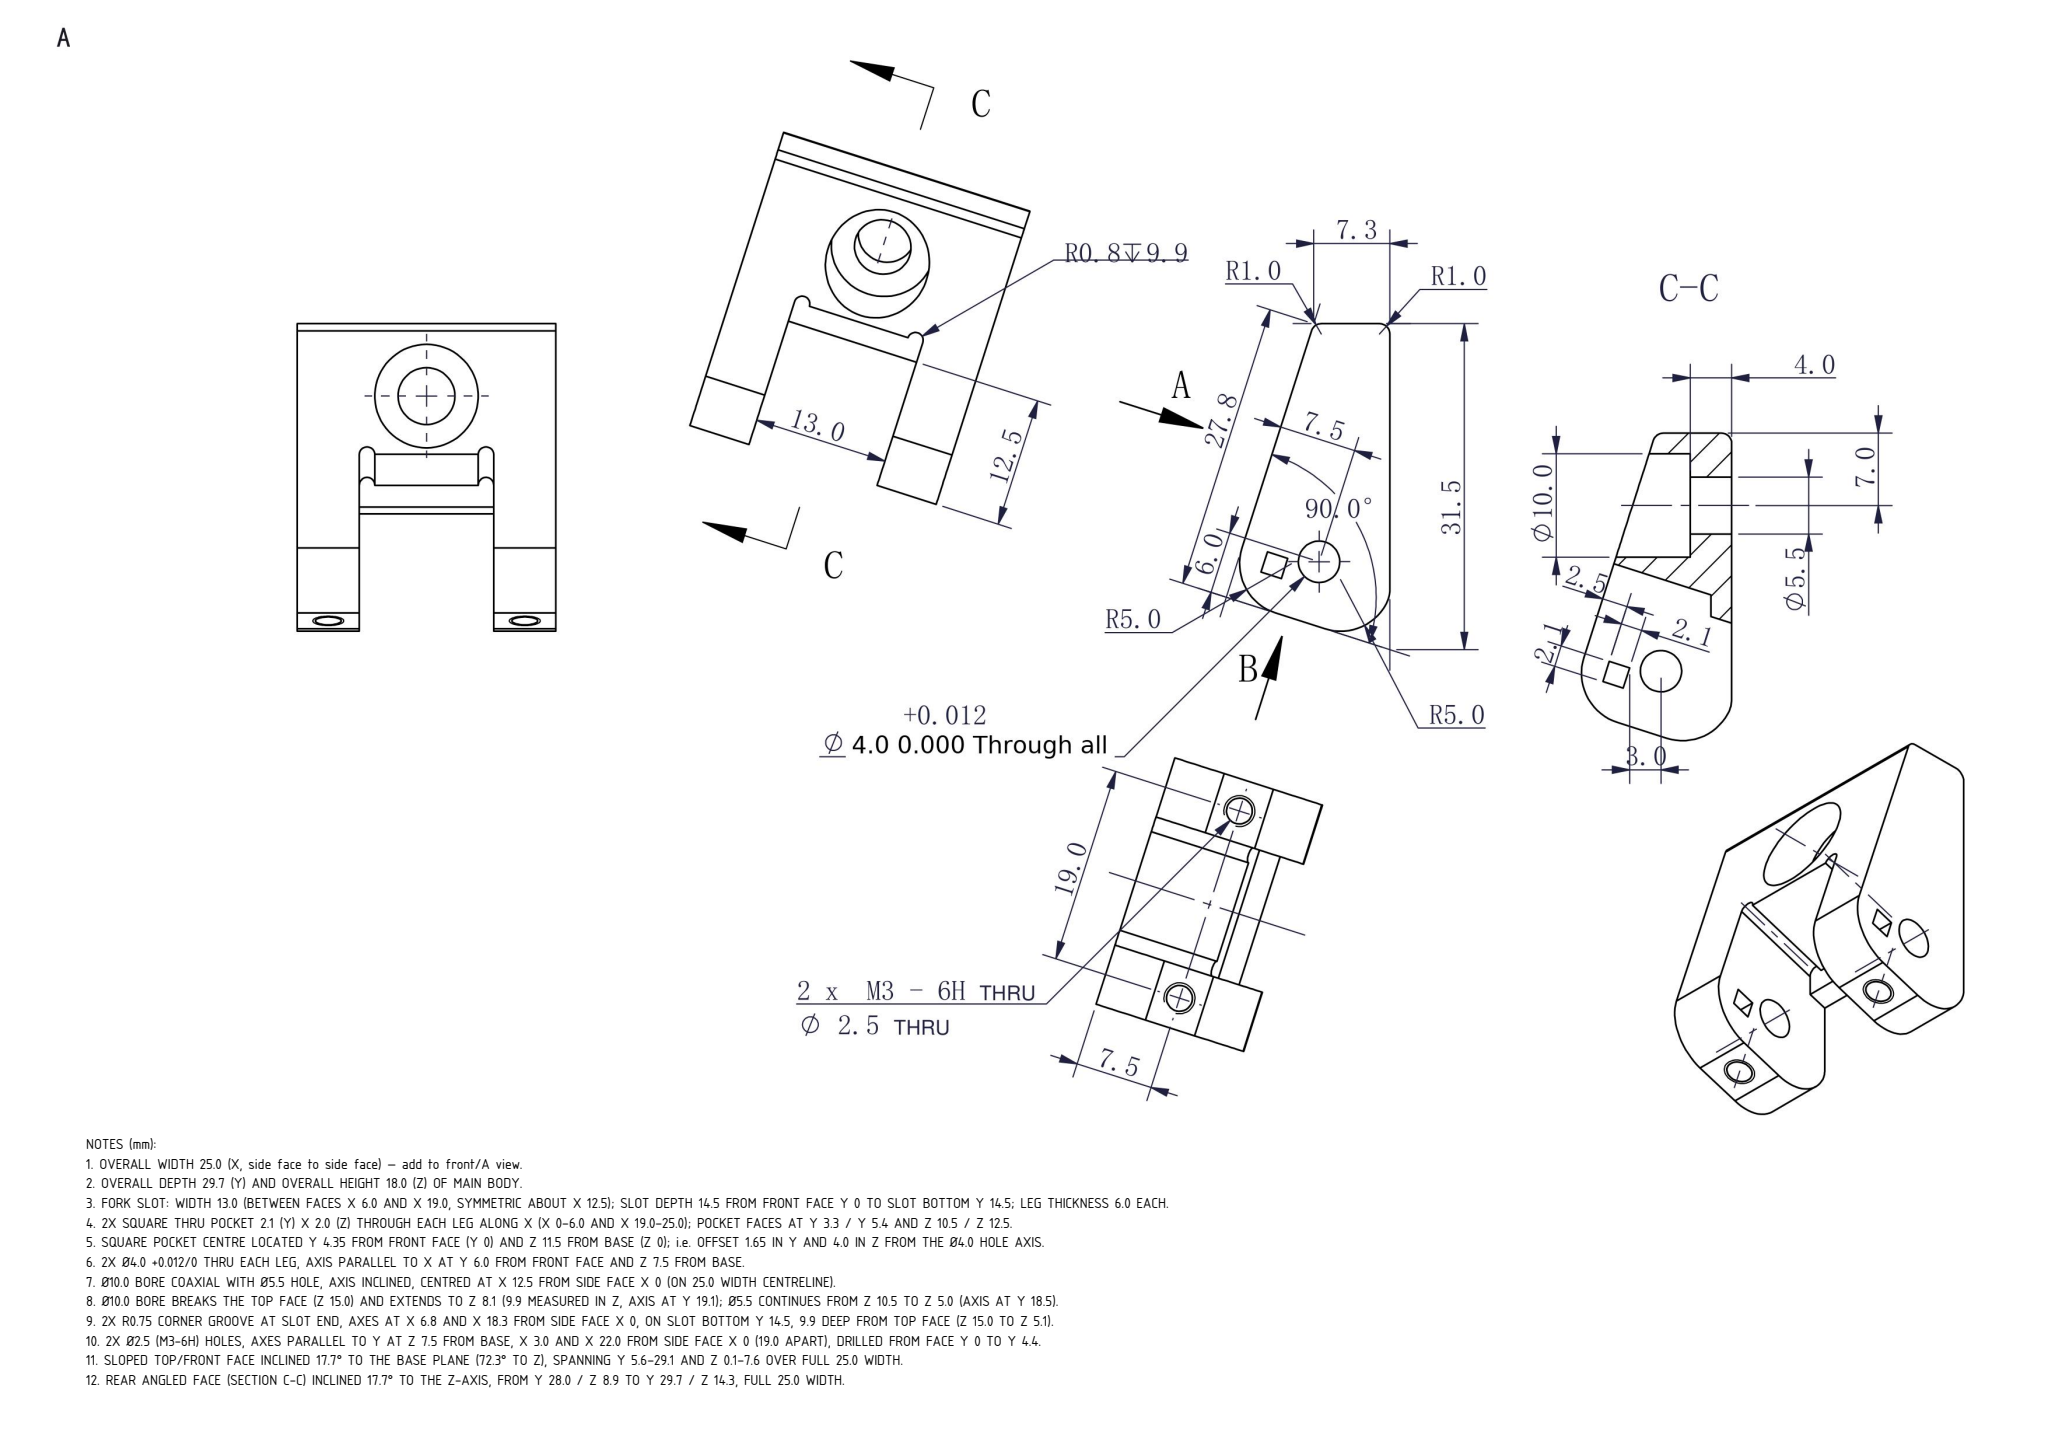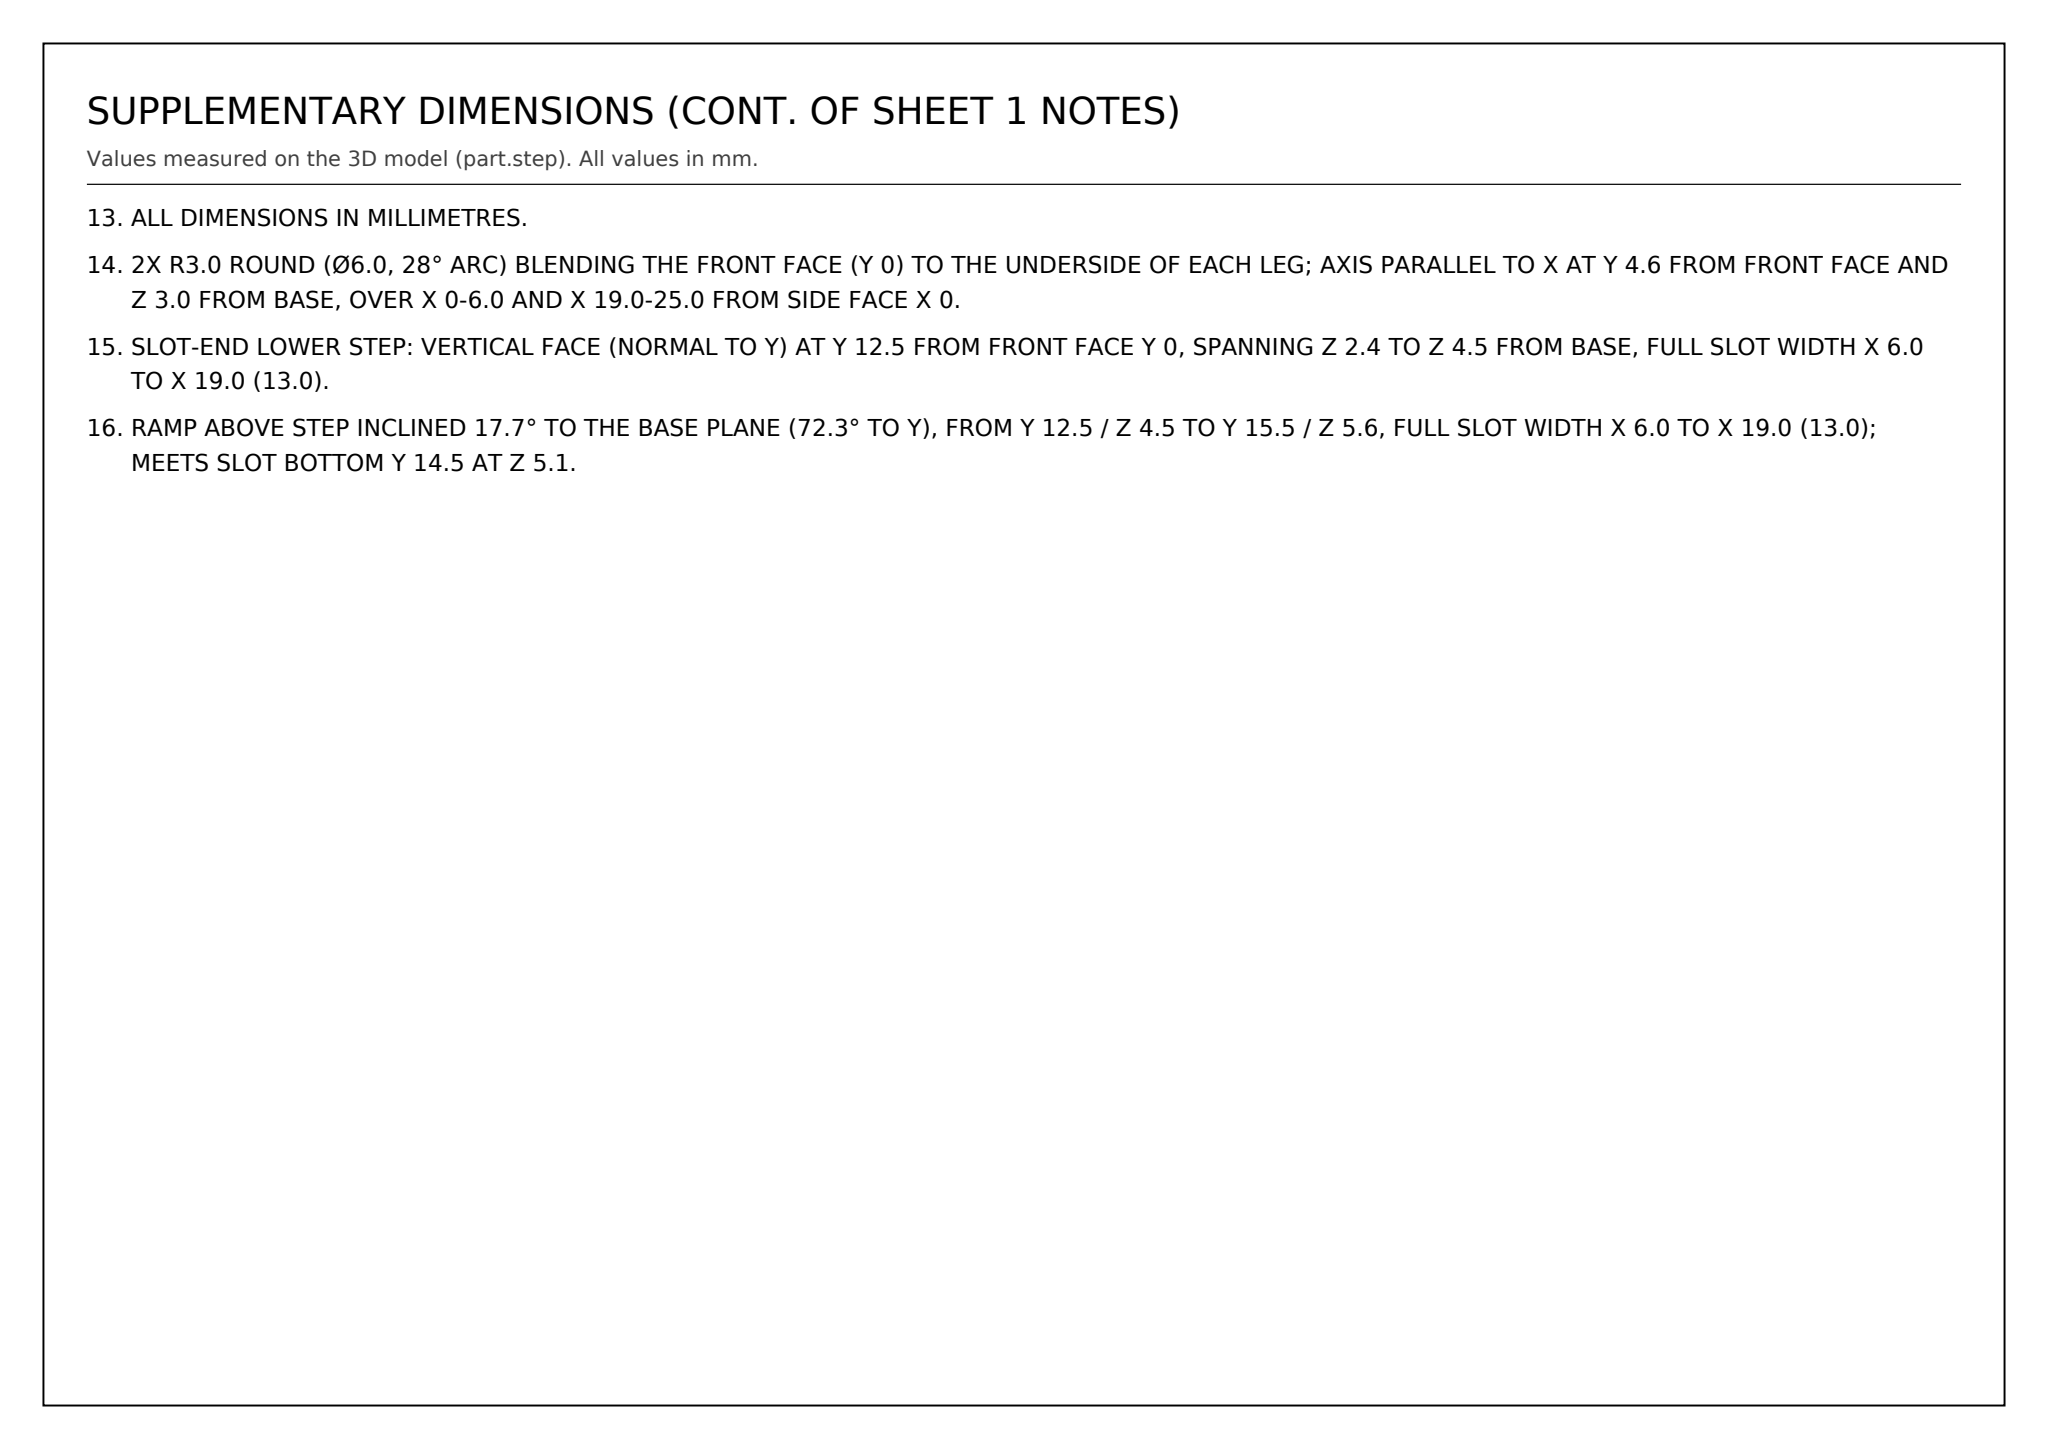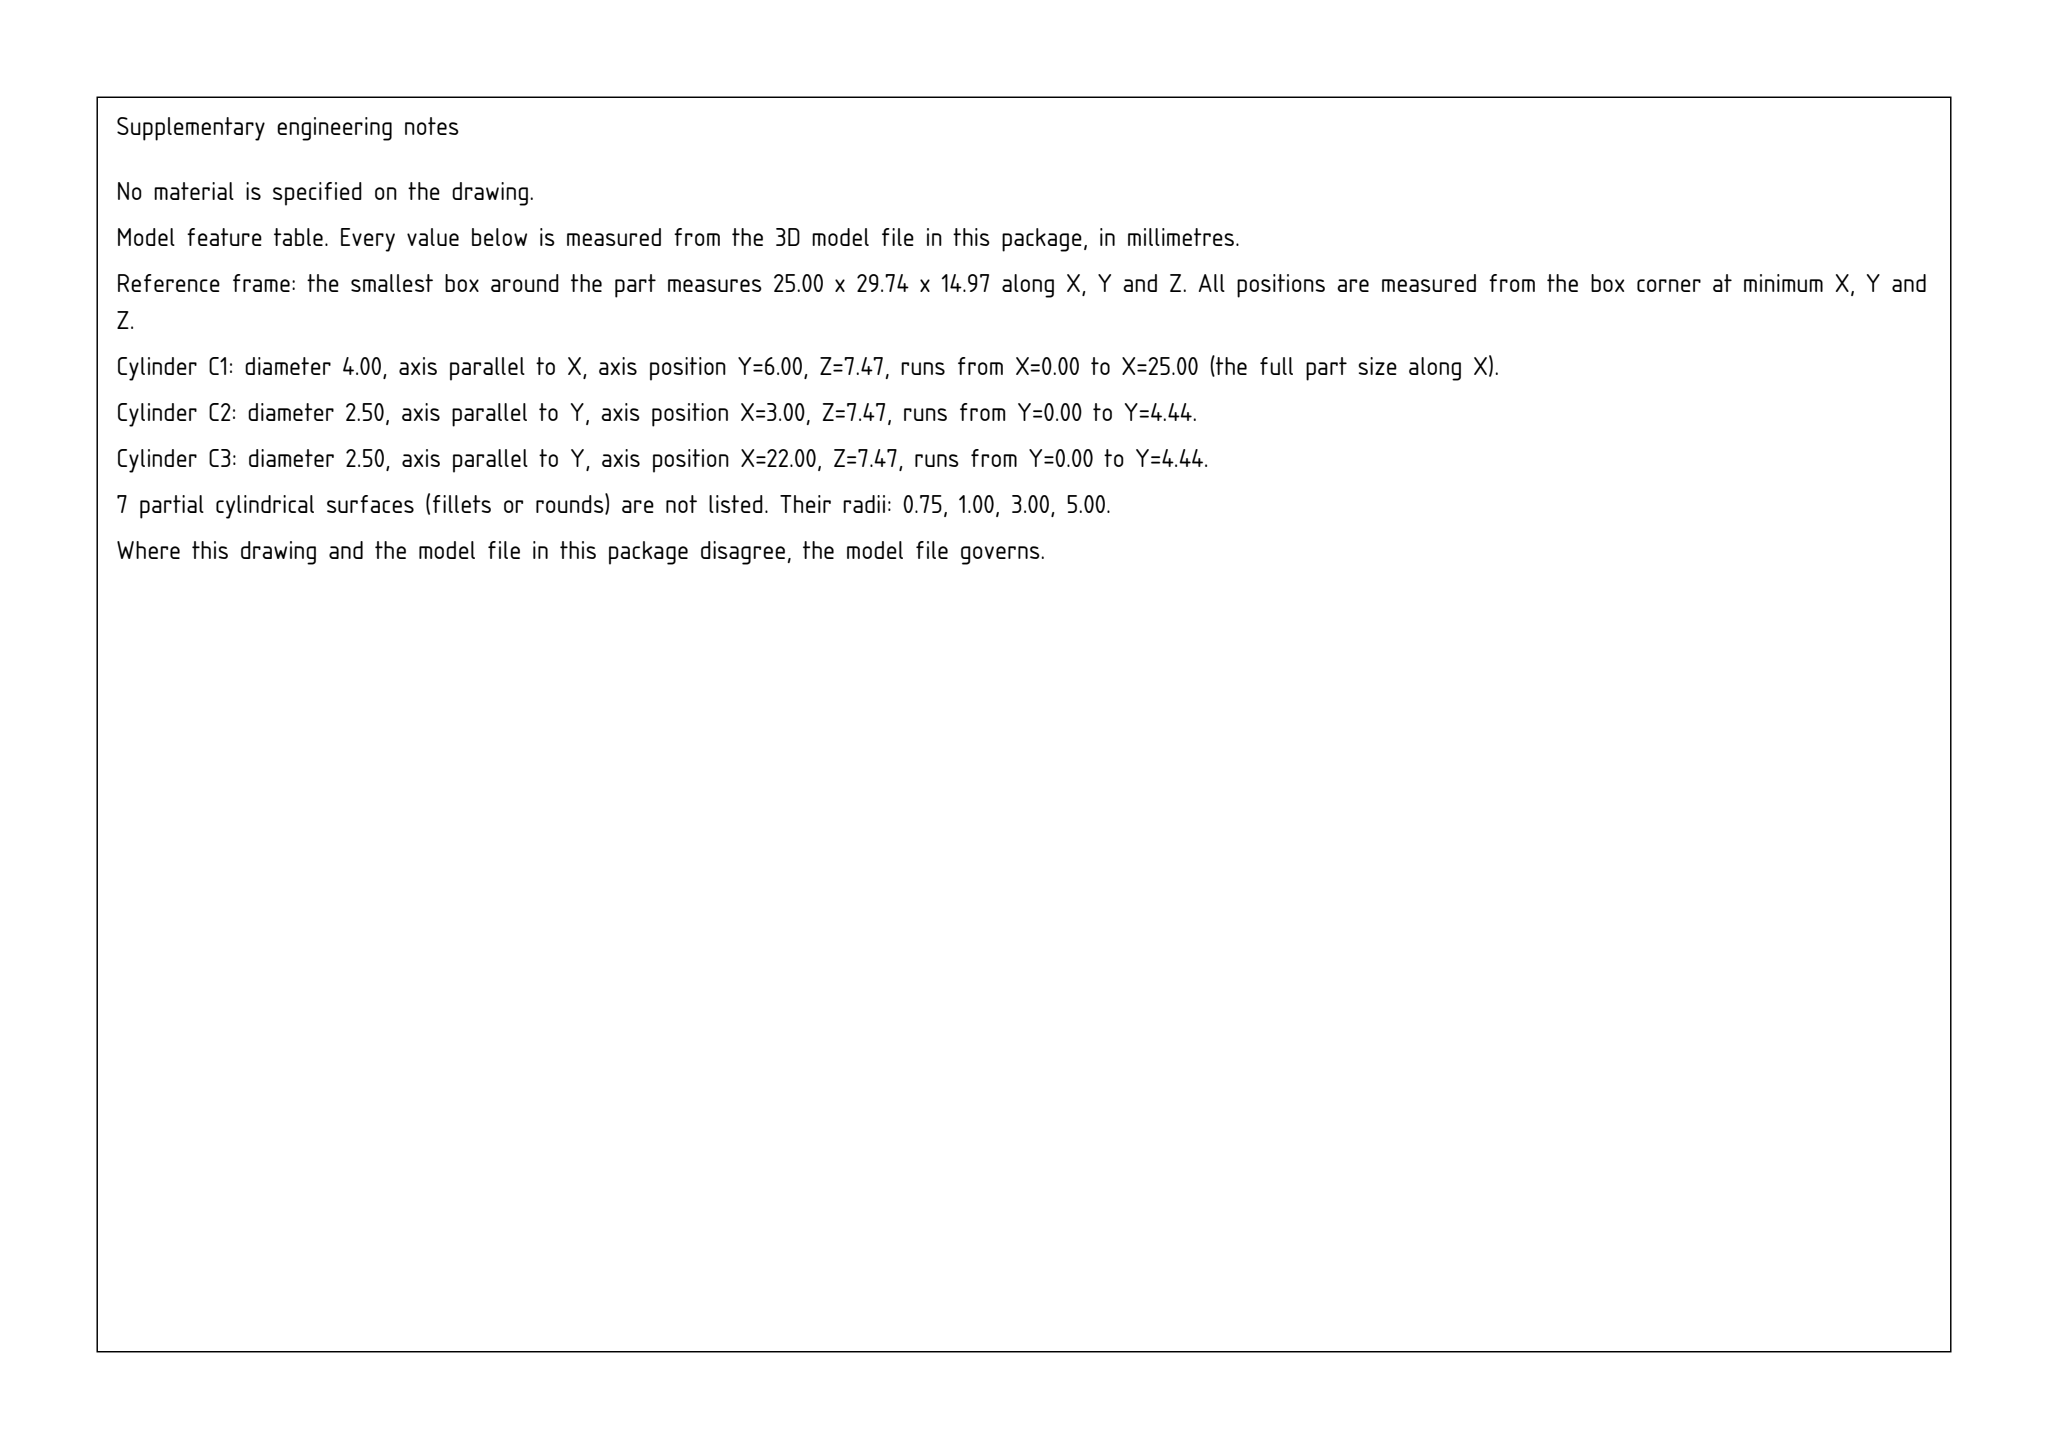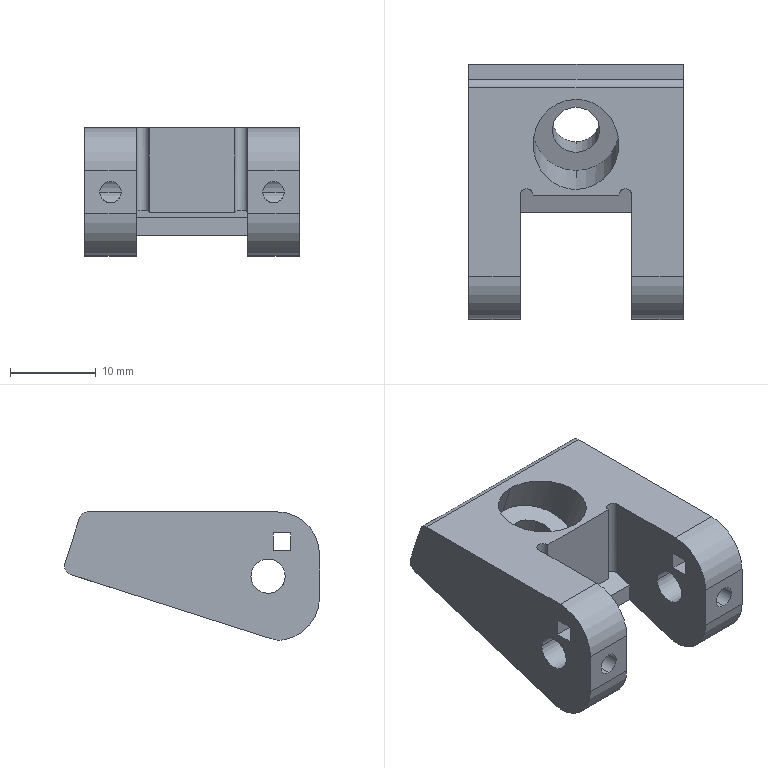Part | SolidWorks | mm | 1 solid | 46 faces | box 25 x 29.74 x 14.97 mm | volume 5039 mm3 | cylinder 25 | plane 21 | commonest cylinder face diameters 10 x6 2.5 x4 6 x4 4 x4 2 x3 5.5 x2 1.5 x2
Drawing notes:
OVERALL WIDTH 25.0 (X, side face to side face) — add to front/A view. | from the solid: bbox_xyz X = 25.0; planes x=0.0 and x=25.0
OVERALL DEPTH 29.7 (Y) AND OVERALL HEIGHT 18.0 (Z) OF MAIN BODY. | from the solid: bbox_xyz = [25.0, 29.743, 18.014]
FORK SLOT: WIDTH 13.0 (BETWEEN FACES X 6.0 AND X 19.0, SYMMETRIC ABOUT X 12.5); SLOT DEPTH 14.5 FROM FRONT FACE Y 0 TO SLOT BOTTOM Y 14.5; LEG THICKNESS 6.0 EACH. | from the solid: axis_planes x=6.0 and x=19.0 (y 0–14.5, z 0–15.0); plane y=14.5 (x 7.5–17.5)
2X SQUARE THRU POCKET 2.1 (Y) X 2.0 (Z) THROUGH EACH LEG ALONG X (X 0–6.0 AND X 19.0–25.0); POCKET FACES AT Y 3.3 / Y 5.4 AND Z 10.5 / Z 12.5. | from the solid: axis_planes y=3.3, y=5.4 (x 0–6 and 19–25, z 10.5–12.5) and z=10.5, z=12.5 (y 3.3–5.4)
SQUARE POCKET CENTRE LOCATED Y 4.35 FROM FRONT FACE (Y 0) AND Z 11.5 FROM BASE (Z 0); i.e. OFFSET 1.65 IN Y AND 4.0 IN Z FROM THE Ø4.0 HOLE AXIS. | from the solid: pocket planes y 3.3/5.4, z 10.5/12.5 vs cylinder dia 4.0 axis at y=6.0, z=7.5
2X Ø4.0 +0.012/0 THRU EACH LEG, AXIS PARALLEL TO X AT Y 6.0 FROM FRONT FACE AND Z 7.5 FROM BASE. | from the solid: hole/bore dia 4.0, axis x, axis_pos [y 6.0, z 7.5], from 0.0 to 6.0 and 19.0 to 25.0
Ø10.0 BORE COAXIAL WITH Ø5.5 HOLE, AXIS INCLINED, CENTRED AT X 12.5 FROM SIDE FACE X 0 (ON 25.0 WIDTH CENTRELINE). | from the solid: hole/bore dia 10.0 and dia 5.5, axis inclined, axis_pos_other_axes x = 12.5
Ø10.0 BORE BREAKS THE TOP FACE (Z 15.0) AND EXTENDS TO Z 8.1 (9.9 MEASURED IN Z, AXIS AT Y 19.1); Ø5.5 CONTINUES FROM Z 10.5 TO Z 5.0 (AXIS AT Y 18.5). | from the solid: hole/bore dia 10.0 from z 8.1 to 18.0 at y 19.1; dia 5.5 from z 5.0 to 10.5 at y 18.5
2X R0.75 CORNER GROOVE AT SLOT END, AXES AT X 6.8 AND X 18.3 FROM SIDE FACE X 0, ON SLOT BOTTOM Y 14.5, 9.9 DEEP FROM TOP FACE (Z 15.0 TO Z 5.1). | from the solid: concave arcs dia 1.5, axis z at (18.3, 14.5) and (6.8, 14.5), from 5.1 to 15.0
2X Ø2.5 (M3-6H) HOLES, AXES PARALLEL TO Y AT Z 7.5 FROM BASE, X 3.0 AND X 22.0 FROM SIDE FACE X 0 (19.0 APART), DRILLED FROM FACE Y 0 TO Y 4.4. | from the solid: hole/bore dia 2.5, axis y, axis_pos (x 3.0, z 7.5) and (x 22.0, z 7.5), from 0.0 to 4.4
SLOPED TOP/FRONT FACE INCLINED 17.7° TO THE BASE PLANE (72.3° TO Z), SPANNING Y 5.6–29.1 AND Z 0.1–7.6 OVER FULL 25.0 WIDTH. | from the solid: inclined_plane angle_to_xyz_axes [90.0, 72.3, 17.7], bbox_from [0.0, 5.6, 0.1], size [25.0, 23.5, 7.5]
REAR ANGLED FACE (SECTION C-C) INCLINED 17.7° TO THE Z-AXIS, FROM Y 28.0 / Z 8.9 TO Y 29.7 / Z 14.3, FULL 25.0 WIDTH. | from the solid: inclined_plane angle_to_xyz_axes [90.0, 17.7, 72.3], bbox_from [0.0, 28.0, 8.9], size [25.0, 1.7, 5.4]
ALL DIMENSIONS IN MILLIMETRES. | from the solid: STEP model facts stated in mm
2X R3.0 ROUND (Ø6.0, 28° ARC) BLENDING THE FRONT FACE (Y 0) TO THE UNDERSIDE OF EACH LEG; AXIS PARALLEL TO X AT Y 4.6 FROM FRONT FACE AND Z 3.0 FROM BASE, OVER X 0-6.0 AND X 19.0-25.0 FROM SIDE FACE X 0. | from the solid: cylinders: convex arc (round/outer radius) dia 6.0, axis x, axis_pos [y 4.6, z 3.0], from 0.0 to 6.0 and from 19.0 to 25.0, arc_deg 28 (2 occurrences)
SLOT-END LOWER STEP: VERTICAL FACE (NORMAL TO Y) AT Y 12.5 FROM FRONT FACE Y 0, SPANNING Z 2.4 TO Z 4.5 FROM BASE, FULL SLOT WIDTH X 6.0 TO X 19.0 (13.0). | from the solid: axis_planes: y-normal plane at offset 12.5, extent x [6.0,19.0], z [2.4,4.5]
RAMP ABOVE STEP INCLINED 17.7° TO THE BASE PLANE (72.3° TO Y), FROM Y 12.5 / Z 4.5 TO Y 15.5 / Z 5.6, FULL SLOT WIDTH X 6.0 TO X 19.0 (13.0); MEETS SLOT BOTTOM Y 14.5 AT Z 5.1. | from the solid: inclined_planes: angle_to_xyz_axes [90.0,72.3,17.7], bbox_from [6.0,12.5,4.5], size [13.0,3.0,1.1]